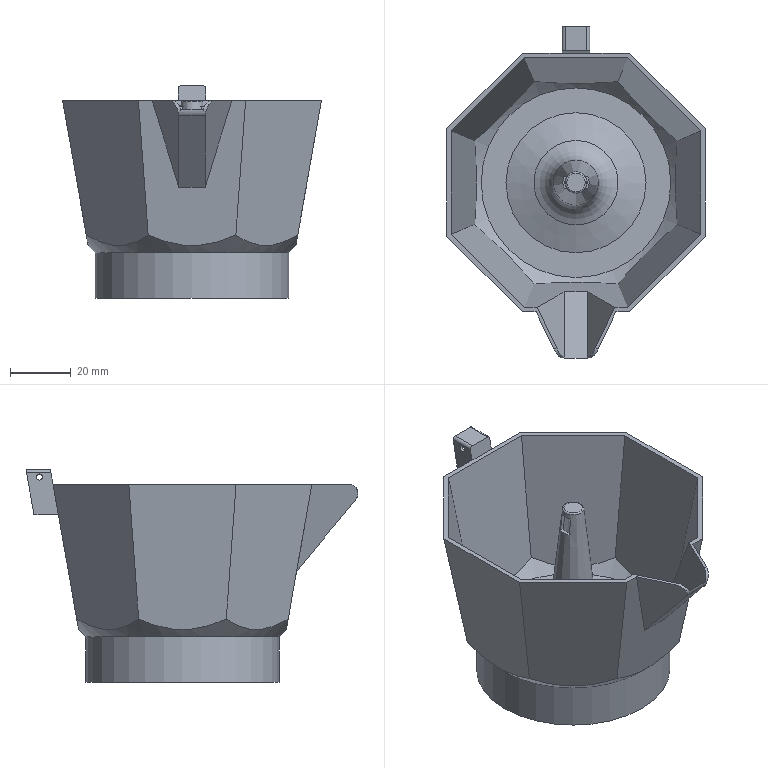Component | NX | MODEL25 | 1 solid | 147 faces | volume 28771 mm3 | cylinder 87 | plane 49 | cone 6 | torus 3 | other 2 | commonest cylinder face diameters 1 x82 2 x2 6 x1 63.5 x1 62 x1